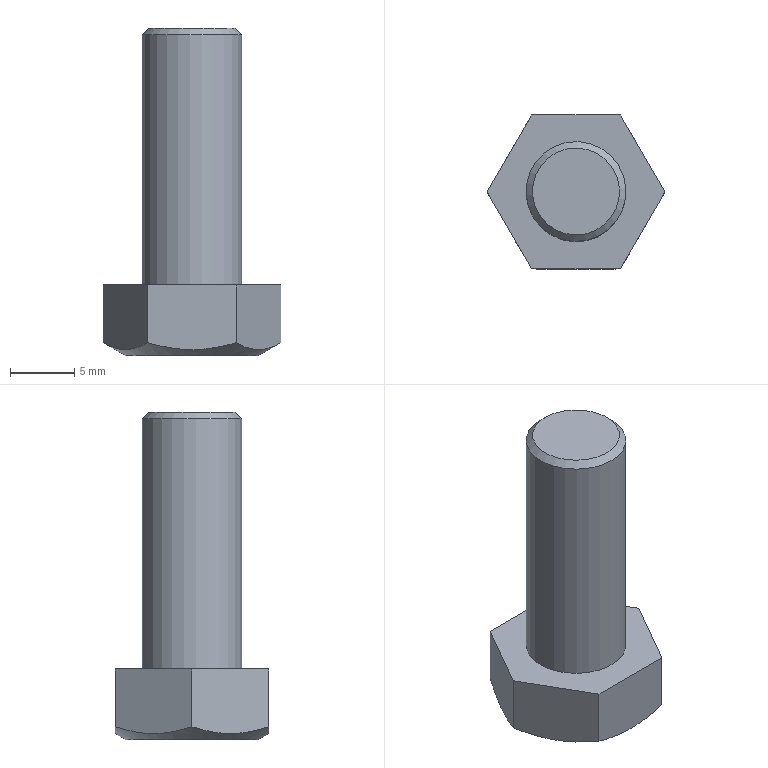Component | NX | BOLT_M8_X_20_2 | 1 solid | 12 faces | box 13.86 x 12 x 25.5 mm | volume 1621 mm3 | plane 9 | cone 2 | cylinder 1 | commonest cylinder face diameters 7.785 x1
STEP:
#1=CARTESIAN_POINT('',(0.,0.,0.));
#2=DIRECTION('',(0.,0.,1.));
#3=DIRECTION('',(1.,0.,0.));
#4=AXIS2_PLACEMENT_3D('',#1,#2,#3);
#5=CARTESIAN_POINT('',(-10.196,-39.311,-58.));
#6=VERTEX_POINT('',#5);
#7=CARTESIAN_POINT('',(-8.5,-36.373,-58.));
#8=DIRECTION('',(0.,0.,1.));
#9=DIRECTION('',(-0.5,-0.866,0.));
#10=AXIS2_PLACEMENT_3D('',#7,#8,#9);
#11=CIRCLE('',#10,3.393);
#12=CARTESIAN_POINT('',(-8.5,-36.373,-58.));
#13=DIRECTION('',(0.,0.,1.));
#14=DIRECTION('',(-0.5,-0.866,0.));
#15=AXIS2_PLACEMENT_3D('',#12,#13,#14);
#16=PLANE('',#15);
#17=CARTESIAN_POINT('',(0.,0.));
#18=DIRECTION('',(1.,-0.));
#19=AXIS2_PLACEMENT_2D('',#17,#18);
#20=CIRCLE('',#19,3.393);
#21=(GEOMETRIC_REPRESENTATION_CONTEXT(2)PARAMETRIC_REPRESENTATION_CONTEXT()REPRESENTATION_CONTEXT('',''));
#22=DEFINITIONAL_REPRESENTATION('',(#20),#21);
#23=PCURVE('',#16,#22);
#24=CARTESIAN_POINT('',(-8.5,-36.373,-58.5));
#25=DIRECTION('',(0.,0.,-1.));
#26=DIRECTION('',(0.5,0.866,0.));
#27=AXIS2_PLACEMENT_3D('',#24,#25,#26);
#28=CONICAL_SURFACE('',#27,3.893,0.7854);
#29=CARTESIAN_POINT('',(9.425,-0.5));
#30=DIRECTION('',(-1.,0.));
#31=VECTOR('',#30,1.);
#32=LINE('',#29,#31);
#33=(GEOMETRIC_REPRESENTATION_CONTEXT(2)PARAMETRIC_REPRESENTATION_CONTEXT()REPRESENTATION_CONTEXT('',''));
#34=DEFINITIONAL_REPRESENTATION('',(#32),#33);
#35=PCURVE('',#28,#34);
#36=SURFACE_CURVE('',#11,(#23,#35),.PCURVE_S1.);
#37=EDGE_CURVE('',#6,#6,#36,.T.);
#38=ORIENTED_EDGE('',*,*,#37,.T.);
#39=EDGE_LOOP('',(#38));
#40=FACE_BOUND('',#39,.T.);
#41=ADVANCED_FACE('',(#40),#16,.T.);
#42=CARTESIAN_POINT('',(-10.446,-39.744,-58.5));
#43=VERTEX_POINT('',#42);
#44=CARTESIAN_POINT('',(-6.554,-33.002,-58.5));
#45=VERTEX_POINT('',#44);
#46=CARTESIAN_POINT('',(-8.5,-36.373,-58.5));
#47=DIRECTION('',(0.,0.,-1.));
#48=DIRECTION('',(-0.5,-0.866,0.));
#49=AXIS2_PLACEMENT_3D('',#46,#47,#48);
#50=CIRCLE('',#49,3.893);
#51=CARTESIAN_POINT('',(-8.5,-36.373,-58.));
#52=DIRECTION('',(0.,0.,-1.));
#53=DIRECTION('',(0.5,0.866,0.));
#54=AXIS2_PLACEMENT_3D('',#51,#52,#53);
#55=CYLINDRICAL_SURFACE('',#54,3.893);
#56=CARTESIAN_POINT('',(3.142,0.5));
#57=DIRECTION('',(1.,0.));
#58=VECTOR('',#57,1.);
#59=LINE('',#56,#58);
#60=(GEOMETRIC_REPRESENTATION_CONTEXT(2)PARAMETRIC_REPRESENTATION_CONTEXT()REPRESENTATION_CONTEXT('',''));
#61=DEFINITIONAL_REPRESENTATION('',(#59),#60);
#62=PCURVE('',#55,#61);
#63=CARTESIAN_POINT('',(3.142,0.));
#64=DIRECTION('',(1.,0.));
#65=VECTOR('',#64,1.);
#66=LINE('',#63,#65);
#67=(GEOMETRIC_REPRESENTATION_CONTEXT(2)PARAMETRIC_REPRESENTATION_CONTEXT()REPRESENTATION_CONTEXT('',''));
#68=DEFINITIONAL_REPRESENTATION('',(#66),#67);
#69=PCURVE('',#28,#68);
#70=SURFACE_CURVE('',#50,(#62,#69),.PCURVE_S1.);
#71=EDGE_CURVE('',#43,#45,#70,.T.);
#72=ORIENTED_EDGE('',*,*,#71,.T.);
#73=CARTESIAN_POINT('',(-6.554,-33.002,-78.));
#74=VERTEX_POINT('',#73);
#75=CARTESIAN_POINT('',(-6.554,-33.002,-58.5));
#76=CARTESIAN_POINT('',(-6.554,-33.002,-78.));
#77=B_SPLINE_CURVE_WITH_KNOTS('',1,(#75,#76),.UNSPECIFIED.,.F.,.F.,(2,2),(0.5,20.),.PIECEWISE_BEZIER_KNOTS.);
#78=CARTESIAN_POINT('',(6.283,0.));
#79=DIRECTION('',(0.,1.));
#80=VECTOR('',#79,1.);
#81=LINE('',#78,#80);
#82=(GEOMETRIC_REPRESENTATION_CONTEXT(2)PARAMETRIC_REPRESENTATION_CONTEXT()REPRESENTATION_CONTEXT('',''));
#83=DEFINITIONAL_REPRESENTATION('',(#81),#82);
#84=PCURVE('',#55,#83);
#85=CARTESIAN_POINT('',(0.,0.));
#86=DIRECTION('',(0.,1.));
#87=VECTOR('',#86,1.);
#88=LINE('',#85,#87);
#89=(GEOMETRIC_REPRESENTATION_CONTEXT(2)PARAMETRIC_REPRESENTATION_CONTEXT()REPRESENTATION_CONTEXT('',''));
#90=DEFINITIONAL_REPRESENTATION('',(#88),#89);
#91=PCURVE('',#55,#90);
#92=SEAM_CURVE('',#77,(#84,#91),.PCURVE_S1.);
#93=EDGE_CURVE('',#45,#74,#92,.T.);
#94=ORIENTED_EDGE('',*,*,#93,.T.);
#95=CARTESIAN_POINT('',(-8.5,-36.373,-78.));
#96=DIRECTION('',(0.,0.,1.));
#97=DIRECTION('',(0.5,0.866,0.));
#98=AXIS2_PLACEMENT_3D('',#95,#96,#97);
#99=CIRCLE('',#98,3.893);
#100=CARTESIAN_POINT('',(6.283,20.));
#101=DIRECTION('',(-1.,0.));
#102=VECTOR('',#101,1.);
#103=LINE('',#100,#102);
#104=(GEOMETRIC_REPRESENTATION_CONTEXT(2)PARAMETRIC_REPRESENTATION_CONTEXT()REPRESENTATION_CONTEXT('',''));
#105=DEFINITIONAL_REPRESENTATION('',(#103),#104);
#106=PCURVE('',#55,#105);
#107=CARTESIAN_POINT('',(-8.5,-36.373,-78.));
#108=DIRECTION('',(0.,0.,1.));
#109=DIRECTION('',(-0.5,-0.866,0.));
#110=AXIS2_PLACEMENT_3D('',#107,#108,#109);
#111=PLANE('',#110);
#112=CARTESIAN_POINT('',(0.,0.));
#113=DIRECTION('',(-1.,0.));
#114=AXIS2_PLACEMENT_2D('',#112,#113);
#115=CIRCLE('',#114,3.893);
#116=(GEOMETRIC_REPRESENTATION_CONTEXT(2)PARAMETRIC_REPRESENTATION_CONTEXT()REPRESENTATION_CONTEXT('',''));
#117=DEFINITIONAL_REPRESENTATION('',(#115),#116);
#118=PCURVE('',#111,#117);
#119=SURFACE_CURVE('',#99,(#106,#118),.PCURVE_S1.);
#120=EDGE_CURVE('',#74,#74,#119,.T.);
#121=ORIENTED_EDGE('',*,*,#120,.T.);
#122=ORIENTED_EDGE('',*,*,#93,.F.);
#123=CARTESIAN_POINT('',(-8.5,-36.373,-58.5));
#124=DIRECTION('',(0.,0.,-1.));
#125=DIRECTION('',(-0.5,-0.866,0.));
#126=AXIS2_PLACEMENT_3D('',#123,#124,#125);
#127=CIRCLE('',#126,3.893);
#128=CARTESIAN_POINT('',(-3.142,0.5));
#129=DIRECTION('',(1.,0.));
#130=VECTOR('',#129,1.);
#131=LINE('',#128,#130);
#132=(GEOMETRIC_REPRESENTATION_CONTEXT(2)PARAMETRIC_REPRESENTATION_CONTEXT()REPRESENTATION_CONTEXT('',''));
#133=DEFINITIONAL_REPRESENTATION('',(#131),#132);
#134=PCURVE('',#55,#133);
#135=CARTESIAN_POINT('',(3.142,0.));
#136=DIRECTION('',(1.,-0.));
#137=VECTOR('',#136,1.);
#138=LINE('',#135,#137);
#139=(GEOMETRIC_REPRESENTATION_CONTEXT(2)PARAMETRIC_REPRESENTATION_CONTEXT()REPRESENTATION_CONTEXT('',''));
#140=DEFINITIONAL_REPRESENTATION('',(#138),#139);
#141=PCURVE('',#28,#140);
#142=SURFACE_CURVE('',#127,(#134,#141),.PCURVE_S1.);
#143=EDGE_CURVE('',#45,#43,#142,.T.);
#144=ORIENTED_EDGE('',*,*,#143,.T.);
#145=EDGE_LOOP('',(#72,#94,#121,#122,#144));
#146=FACE_BOUND('',#145,.T.);
#147=ADVANCED_FACE('',(#146),#55,.T.);
#148=CARTESIAN_POINT('',(-5.036,-30.373,-82.5));
#149=VERTEX_POINT('',#148);
#150=CARTESIAN_POINT('',(-1.572,-36.373,-82.5));
#151=VERTEX_POINT('',#150);
#152=CARTESIAN_POINT('',(-5.036,-30.373,-82.5));
#153=CARTESIAN_POINT('',(-4.47,-31.353,-82.827));
#154=CARTESIAN_POINT('',(-3.896,-32.347,-83.035));
#155=CARTESIAN_POINT('',(-2.718,-34.388,-83.037));
#156=CARTESIAN_POINT('',(-2.138,-35.392,-82.827));
#157=CARTESIAN_POINT('',(-1.572,-36.373,-82.5));
#158=B_SPLINE_CURVE_WITH_KNOTS('',3,(#152,#153,#154,#155,#156,#157),.UNSPECIFIED.,.F.,.F.,(4,2,4),(0.,0.5,1.),.UNSPECIFIED.);
#159=CARTESIAN_POINT('',(-1.572,-36.373,-83.5));
#160=DIRECTION('',(0.866,0.5,0.));
#161=DIRECTION('',(0.5,-0.866,0.));
#162=AXIS2_PLACEMENT_3D('',#159,#160,#161);
#163=PLANE('',#162);
#164=CARTESIAN_POINT('',(-6.928,-1.));
#165=CARTESIAN_POINT('',(-5.797,-0.6734));
#166=CARTESIAN_POINT('',(-4.649,-0.4649));
#167=CARTESIAN_POINT('',(-2.293,-0.4634));
#168=CARTESIAN_POINT('',(-1.133,-0.673));
#169=CARTESIAN_POINT('',(0.,-1.));
#170=B_SPLINE_CURVE_WITH_KNOTS('',3,(#164,#165,#166,#167,#168,#169),.UNSPECIFIED.,.F.,.F.,(4,2,4),(0.,0.5,1.),.UNSPECIFIED.);
#171=(GEOMETRIC_REPRESENTATION_CONTEXT(2)PARAMETRIC_REPRESENTATION_CONTEXT()REPRESENTATION_CONTEXT('',''));
#172=DEFINITIONAL_REPRESENTATION('',(#170),#171);
#173=PCURVE('',#163,#172);
#174=CARTESIAN_POINT('',(-8.5,-36.373,-83.5));
#175=DIRECTION('',(0.,0.,1.));
#176=DIRECTION('',(-0.5,-0.866,0.));
#177=AXIS2_PLACEMENT_3D('',#174,#175,#176);
#178=CONICAL_SURFACE('',#177,5.196,1.047);
#179=CARTESIAN_POINT('',(3.142,1.));
#180=CARTESIAN_POINT('',(3.129,0.9703));
#181=CARTESIAN_POINT('',(3.102,0.9129));
#182=CARTESIAN_POINT('',(3.061,0.8328));
#183=CARTESIAN_POINT('',(3.018,0.7594));
#184=CARTESIAN_POINT('',(2.973,0.6931));
#185=CARTESIAN_POINT('',(2.926,0.6342));
#186=CARTESIAN_POINT('',(2.878,0.5834));
#187=CARTESIAN_POINT('',(2.828,0.5409));
#188=CARTESIAN_POINT('',(2.777,0.5072));
#189=CARTESIAN_POINT('',(2.725,0.4827));
#190=CARTESIAN_POINT('',(2.673,0.4677));
#191=CARTESIAN_POINT('',(2.619,0.4624));
#192=CARTESIAN_POINT('',(2.566,0.4673));
#193=CARTESIAN_POINT('',(2.513,0.4819));
#194=CARTESIAN_POINT('',(2.46,0.5062));
#195=CARTESIAN_POINT('',(2.409,0.5398));
#196=CARTESIAN_POINT('',(2.359,0.5823));
#197=CARTESIAN_POINT('',(2.311,0.6332));
#198=CARTESIAN_POINT('',(2.264,0.6922));
#199=CARTESIAN_POINT('',(2.218,0.7588));
#200=CARTESIAN_POINT('',(2.175,0.8325));
#201=CARTESIAN_POINT('',(2.134,0.9127));
#202=CARTESIAN_POINT('',(2.107,0.9703));
#203=CARTESIAN_POINT('',(2.094,1.));
#204=B_SPLINE_CURVE_WITH_KNOTS('',3,(#179,#180,#181,#182,#183,#184,#185,#186,#187,#188,#189,#190,#191,#192,#193,#194,#195,#196,#197,#198,#199,#200,#201,#202,#203),.UNSPECIFIED.,.F.,.F.,(4,1,1,1,1,1,1,1,1,1,1,1,1,1,1,1,1,1,1,1,1,1,4),(0.,0.04545,0.09091,0.1364,0.1818,0.2273,0.2727,0.3182,0.3636,0.4091,0.4545,0.5,0.5455,0.5909,0.6364,0.6818,0.7273,0.7727,0.8182,0.8636,0.9091,0.9545,1.),.QUASI_UNIFORM_KNOTS.);
#205=(GEOMETRIC_REPRESENTATION_CONTEXT(2)PARAMETRIC_REPRESENTATION_CONTEXT()REPRESENTATION_CONTEXT('',''));
#206=DEFINITIONAL_REPRESENTATION('',(#204),#205);
#207=PCURVE('',#178,#206);
#208=SURFACE_CURVE('',#158,(#173,#207),.PCURVE_S1.);
#209=EDGE_CURVE('',#149,#151,#208,.T.);
#210=ORIENTED_EDGE('',*,*,#209,.F.);
#211=CARTESIAN_POINT('',(-5.036,-30.373,-78.));
#212=VERTEX_POINT('',#211);
#213=CARTESIAN_POINT('',(-5.036,-30.373,-83.5));
#214=DIRECTION('',(0.,0.,1.));
#215=VECTOR('',#214,1.);
#216=LINE('',#213,#215);
#217=CARTESIAN_POINT('',(-6.928,0.));
#218=DIRECTION('',(0.,-1.));
#219=VECTOR('',#218,1.);
#220=LINE('',#217,#219);
#221=(GEOMETRIC_REPRESENTATION_CONTEXT(2)PARAMETRIC_REPRESENTATION_CONTEXT()REPRESENTATION_CONTEXT('',''));
#222=DEFINITIONAL_REPRESENTATION('',(#220),#221);
#223=PCURVE('',#163,#222);
#224=CARTESIAN_POINT('',(-5.036,-30.373,-83.5));
#225=DIRECTION('',(0.,1.,0.));
#226=DIRECTION('',(1.,-0.,0.));
#227=AXIS2_PLACEMENT_3D('',#224,#225,#226);
#228=PLANE('',#227);
#229=CARTESIAN_POINT('',(0.,0.));
#230=DIRECTION('',(0.,-1.));
#231=VECTOR('',#230,1.);
#232=LINE('',#229,#231);
#233=(GEOMETRIC_REPRESENTATION_CONTEXT(2)PARAMETRIC_REPRESENTATION_CONTEXT()REPRESENTATION_CONTEXT('',''));
#234=DEFINITIONAL_REPRESENTATION('',(#232),#233);
#235=PCURVE('',#228,#234);
#236=SURFACE_CURVE('',#216,(#223,#235),.PCURVE_S1.);
#237=EDGE_CURVE('',#149,#212,#236,.T.);
#238=ORIENTED_EDGE('',*,*,#237,.T.);
#239=CARTESIAN_POINT('',(-1.572,-36.373,-78.));
#240=VERTEX_POINT('',#239);
#241=CARTESIAN_POINT('',(-1.572,-36.373,-78.));
#242=DIRECTION('',(-0.5,0.866,0.));
#243=VECTOR('',#242,1.);
#244=LINE('',#241,#243);
#245=CARTESIAN_POINT('',(0.,-5.5));
#246=DIRECTION('',(-1.,0.));
#247=VECTOR('',#246,1.);
#248=LINE('',#245,#247);
#249=(GEOMETRIC_REPRESENTATION_CONTEXT(2)PARAMETRIC_REPRESENTATION_CONTEXT()REPRESENTATION_CONTEXT('',''));
#250=DEFINITIONAL_REPRESENTATION('',(#248),#249);
#251=PCURVE('',#163,#250);
#252=CARTESIAN_POINT('',(-3.464,6.));
#253=DIRECTION('',(-0.5,-0.866));
#254=VECTOR('',#253,1.);
#255=LINE('',#252,#254);
#256=(GEOMETRIC_REPRESENTATION_CONTEXT(2)PARAMETRIC_REPRESENTATION_CONTEXT()REPRESENTATION_CONTEXT('',''));
#257=DEFINITIONAL_REPRESENTATION('',(#255),#256);
#258=PCURVE('',#111,#257);
#259=SURFACE_CURVE('',#244,(#251,#258),.PCURVE_S1.);
#260=EDGE_CURVE('',#240,#212,#259,.T.);
#261=ORIENTED_EDGE('',*,*,#260,.F.);
#262=CARTESIAN_POINT('',(-1.572,-36.373,-83.5));
#263=DIRECTION('',(0.,0.,1.));
#264=VECTOR('',#263,1.);
#265=LINE('',#262,#264);
#266=CARTESIAN_POINT('',(0.,0.));
#267=DIRECTION('',(0.,-1.));
#268=VECTOR('',#267,1.);
#269=LINE('',#266,#268);
#270=(GEOMETRIC_REPRESENTATION_CONTEXT(2)PARAMETRIC_REPRESENTATION_CONTEXT()REPRESENTATION_CONTEXT('',''));
#271=DEFINITIONAL_REPRESENTATION('',(#269),#270);
#272=PCURVE('',#163,#271);
#273=CARTESIAN_POINT('',(-5.036,-42.373,-83.5));
#274=DIRECTION('',(0.866,-0.5,0.));
#275=DIRECTION('',(0.,0.,-1.));
#276=AXIS2_PLACEMENT_3D('',#273,#274,#275);
#277=PLANE('',#276);
#278=CARTESIAN_POINT('',(0.,6.928));
#279=DIRECTION('',(-1.,0.));
#280=VECTOR('',#279,1.);
#281=LINE('',#278,#280);
#282=(GEOMETRIC_REPRESENTATION_CONTEXT(2)PARAMETRIC_REPRESENTATION_CONTEXT()REPRESENTATION_CONTEXT('',''));
#283=DEFINITIONAL_REPRESENTATION('',(#281),#282);
#284=PCURVE('',#277,#283);
#285=SURFACE_CURVE('',#265,(#272,#284),.PCURVE_S1.);
#286=EDGE_CURVE('',#151,#240,#285,.T.);
#287=ORIENTED_EDGE('',*,*,#286,.F.);
#288=EDGE_LOOP('',(#210,#238,#261,#287));
#289=FACE_BOUND('',#288,.T.);
#290=ADVANCED_FACE('',(#289),#163,.T.);
#291=CARTESIAN_POINT('',(-11.964,-30.373,-82.5));
#292=VERTEX_POINT('',#291);
#293=CARTESIAN_POINT('',(-11.964,-30.373,-82.5));
#294=CARTESIAN_POINT('',(-10.833,-30.373,-82.827));
#295=CARTESIAN_POINT('',(-9.685,-30.373,-83.035));
#296=CARTESIAN_POINT('',(-7.329,-30.373,-83.037));
#297=CARTESIAN_POINT('',(-6.169,-30.373,-82.827));
#298=CARTESIAN_POINT('',(-5.036,-30.373,-82.5));
#299=B_SPLINE_CURVE_WITH_KNOTS('',3,(#293,#294,#295,#296,#297,#298),.UNSPECIFIED.,.F.,.F.,(4,2,4),(0.,0.5,1.),.UNSPECIFIED.);
#300=CARTESIAN_POINT('',(-6.928,-1.));
#301=CARTESIAN_POINT('',(-5.797,-0.6734));
#302=CARTESIAN_POINT('',(-4.649,-0.4649));
#303=CARTESIAN_POINT('',(-2.293,-0.4634));
#304=CARTESIAN_POINT('',(-1.133,-0.673));
#305=CARTESIAN_POINT('',(0.,-1.));
#306=B_SPLINE_CURVE_WITH_KNOTS('',3,(#300,#301,#302,#303,#304,#305),.UNSPECIFIED.,.F.,.F.,(4,2,4),(0.,0.5,1.),.UNSPECIFIED.);
#307=(GEOMETRIC_REPRESENTATION_CONTEXT(2)PARAMETRIC_REPRESENTATION_CONTEXT()REPRESENTATION_CONTEXT('',''));
#308=DEFINITIONAL_REPRESENTATION('',(#306),#307);
#309=PCURVE('',#228,#308);
#310=CARTESIAN_POINT('',(4.189,1.));
#311=CARTESIAN_POINT('',(4.176,0.9703));
#312=CARTESIAN_POINT('',(4.15,0.9129));
#313=CARTESIAN_POINT('',(4.108,0.8328));
#314=CARTESIAN_POINT('',(4.065,0.7594));
#315=CARTESIAN_POINT('',(4.02,0.6931));
#316=CARTESIAN_POINT('',(3.974,0.6342));
#317=CARTESIAN_POINT('',(3.925,0.5834));
#318=CARTESIAN_POINT('',(3.876,0.5409));
#319=CARTESIAN_POINT('',(3.825,0.5072));
#320=CARTESIAN_POINT('',(3.773,0.4827));
#321=CARTESIAN_POINT('',(3.72,0.4677));
#322=CARTESIAN_POINT('',(3.666,0.4624));
#323=CARTESIAN_POINT('',(3.613,0.4673));
#324=CARTESIAN_POINT('',(3.56,0.4819));
#325=CARTESIAN_POINT('',(3.507,0.5062));
#326=CARTESIAN_POINT('',(3.456,0.5398));
#327=CARTESIAN_POINT('',(3.406,0.5823));
#328=CARTESIAN_POINT('',(3.358,0.6332));
#329=CARTESIAN_POINT('',(3.311,0.6922));
#330=CARTESIAN_POINT('',(3.266,0.7588));
#331=CARTESIAN_POINT('',(3.222,0.8325));
#332=CARTESIAN_POINT('',(3.181,0.9127));
#333=CARTESIAN_POINT('',(3.154,0.9703));
#334=CARTESIAN_POINT('',(3.142,1.));
#335=B_SPLINE_CURVE_WITH_KNOTS('',3,(#310,#311,#312,#313,#314,#315,#316,#317,#318,#319,#320,#321,#322,#323,#324,#325,#326,#327,#328,#329,#330,#331,#332,#333,#334),.UNSPECIFIED.,.F.,.F.,(4,1,1,1,1,1,1,1,1,1,1,1,1,1,1,1,1,1,1,1,1,1,4),(0.,0.04545,0.09091,0.1364,0.1818,0.2273,0.2727,0.3182,0.3636,0.4091,0.4545,0.5,0.5455,0.5909,0.6364,0.6818,0.7273,0.7727,0.8182,0.8636,0.9091,0.9545,1.),.QUASI_UNIFORM_KNOTS.);
#336=(GEOMETRIC_REPRESENTATION_CONTEXT(2)PARAMETRIC_REPRESENTATION_CONTEXT()REPRESENTATION_CONTEXT('',''));
#337=DEFINITIONAL_REPRESENTATION('',(#335),#336);
#338=PCURVE('',#178,#337);
#339=SURFACE_CURVE('',#299,(#309,#338),.PCURVE_S1.);
#340=EDGE_CURVE('',#292,#149,#339,.T.);
#341=ORIENTED_EDGE('',*,*,#340,.F.);
#342=CARTESIAN_POINT('',(-11.964,-30.373,-78.));
#343=VERTEX_POINT('',#342);
#344=CARTESIAN_POINT('',(-11.964,-30.373,-83.5));
#345=DIRECTION('',(0.,0.,1.));
#346=VECTOR('',#345,1.);
#347=LINE('',#344,#346);
#348=CARTESIAN_POINT('',(-6.928,0.));
#349=DIRECTION('',(0.,-1.));
#350=VECTOR('',#349,1.);
#351=LINE('',#348,#350);
#352=(GEOMETRIC_REPRESENTATION_CONTEXT(2)PARAMETRIC_REPRESENTATION_CONTEXT()REPRESENTATION_CONTEXT('',''));
#353=DEFINITIONAL_REPRESENTATION('',(#351),#352);
#354=PCURVE('',#228,#353);
#355=CARTESIAN_POINT('',(-11.964,-30.373,-83.5));
#356=DIRECTION('',(-0.866,0.5,0.));
#357=DIRECTION('',(0.5,0.866,0.));
#358=AXIS2_PLACEMENT_3D('',#355,#356,#357);
#359=PLANE('',#358);
#360=CARTESIAN_POINT('',(0.,0.));
#361=DIRECTION('',(0.,-1.));
#362=VECTOR('',#361,1.);
#363=LINE('',#360,#362);
#364=(GEOMETRIC_REPRESENTATION_CONTEXT(2)PARAMETRIC_REPRESENTATION_CONTEXT()REPRESENTATION_CONTEXT('',''));
#365=DEFINITIONAL_REPRESENTATION('',(#363),#364);
#366=PCURVE('',#359,#365);
#367=SURFACE_CURVE('',#347,(#354,#366),.PCURVE_S1.);
#368=EDGE_CURVE('',#292,#343,#367,.T.);
#369=ORIENTED_EDGE('',*,*,#368,.T.);
#370=CARTESIAN_POINT('',(-5.036,-30.373,-78.));
#371=DIRECTION('',(-1.,0.,0.));
#372=VECTOR('',#371,1.);
#373=LINE('',#370,#372);
#374=CARTESIAN_POINT('',(0.,-5.5));
#375=DIRECTION('',(-1.,0.));
#376=VECTOR('',#375,1.);
#377=LINE('',#374,#376);
#378=(GEOMETRIC_REPRESENTATION_CONTEXT(2)PARAMETRIC_REPRESENTATION_CONTEXT()REPRESENTATION_CONTEXT('',''));
#379=DEFINITIONAL_REPRESENTATION('',(#377),#378);
#380=PCURVE('',#228,#379);
#381=CARTESIAN_POINT('',(-6.928,-0.));
#382=DIRECTION('',(0.5,-0.866));
#383=VECTOR('',#382,1.);
#384=LINE('',#381,#383);
#385=(GEOMETRIC_REPRESENTATION_CONTEXT(2)PARAMETRIC_REPRESENTATION_CONTEXT()REPRESENTATION_CONTEXT('',''));
#386=DEFINITIONAL_REPRESENTATION('',(#384),#385);
#387=PCURVE('',#111,#386);
#388=SURFACE_CURVE('',#373,(#380,#387),.PCURVE_S1.);
#389=EDGE_CURVE('',#212,#343,#388,.T.);
#390=ORIENTED_EDGE('',*,*,#389,.F.);
#391=ORIENTED_EDGE('',*,*,#237,.F.);
#392=EDGE_LOOP('',(#341,#369,#390,#391));
#393=FACE_BOUND('',#392,.T.);
#394=ADVANCED_FACE('',(#393),#228,.T.);
#395=CARTESIAN_POINT('',(-15.428,-36.373,-82.5));
#396=VERTEX_POINT('',#395);
#397=CARTESIAN_POINT('',(-15.428,-36.373,-82.5));
#398=CARTESIAN_POINT('',(-14.865,-35.397,-82.825));
#399=CARTESIAN_POINT('',(-14.281,-34.386,-83.036));
#400=CARTESIAN_POINT('',(-13.11,-32.358,-83.036));
#401=CARTESIAN_POINT('',(-12.524,-31.343,-82.823));
#402=CARTESIAN_POINT('',(-11.964,-30.373,-82.5));
#403=B_SPLINE_CURVE_WITH_KNOTS('',3,(#397,#398,#399,#400,#401,#402),.UNSPECIFIED.,.F.,.F.,(4,2,4),(0.,0.5,1.),.UNSPECIFIED.);
#404=CARTESIAN_POINT('',(-6.928,-1.));
#405=CARTESIAN_POINT('',(-5.801,-0.6747));
#406=CARTESIAN_POINT('',(-4.634,-0.464));
#407=CARTESIAN_POINT('',(-2.292,-0.4642));
#408=CARTESIAN_POINT('',(-1.12,-0.6767));
#409=CARTESIAN_POINT('',(0.,-1.));
#410=B_SPLINE_CURVE_WITH_KNOTS('',3,(#404,#405,#406,#407,#408,#409),.UNSPECIFIED.,.F.,.F.,(4,2,4),(0.,0.5,1.),.UNSPECIFIED.);
#411=(GEOMETRIC_REPRESENTATION_CONTEXT(2)PARAMETRIC_REPRESENTATION_CONTEXT()REPRESENTATION_CONTEXT('',''));
#412=DEFINITIONAL_REPRESENTATION('',(#410),#411);
#413=PCURVE('',#359,#412);
#414=CARTESIAN_POINT('',(5.236,1.));
#415=CARTESIAN_POINT('',(5.223,0.9704));
#416=CARTESIAN_POINT('',(5.197,0.9131));
#417=CARTESIAN_POINT('',(5.156,0.833));
#418=CARTESIAN_POINT('',(5.112,0.7594));
#419=CARTESIAN_POINT('',(5.067,0.6928));
#420=CARTESIAN_POINT('',(5.02,0.6338));
#421=CARTESIAN_POINT('',(4.972,0.5827));
#422=CARTESIAN_POINT('',(4.922,0.5402));
#423=CARTESIAN_POINT('',(4.87,0.5065));
#424=CARTESIAN_POINT('',(4.818,0.4822));
#425=CARTESIAN_POINT('',(4.765,0.4674));
#426=CARTESIAN_POINT('',(4.712,0.4624));
#427=CARTESIAN_POINT('',(4.659,0.4675));
#428=CARTESIAN_POINT('',(4.606,0.4823));
#429=CARTESIAN_POINT('',(4.554,0.5068));
#430=CARTESIAN_POINT('',(4.503,0.5406));
#431=CARTESIAN_POINT('',(4.453,0.5833));
#432=CARTESIAN_POINT('',(4.404,0.6345));
#433=CARTESIAN_POINT('',(4.357,0.6936));
#434=CARTESIAN_POINT('',(4.312,0.7602));
#435=CARTESIAN_POINT('',(4.269,0.8337));
#436=CARTESIAN_POINT('',(4.228,0.9136));
#437=CARTESIAN_POINT('',(4.202,0.9706));
#438=CARTESIAN_POINT('',(4.189,1.));
#439=B_SPLINE_CURVE_WITH_KNOTS('',3,(#414,#415,#416,#417,#418,#419,#420,#421,#422,#423,#424,#425,#426,#427,#428,#429,#430,#431,#432,#433,#434,#435,#436,#437,#438),.UNSPECIFIED.,.F.,.F.,(4,1,1,1,1,1,1,1,1,1,1,1,1,1,1,1,1,1,1,1,1,1,4),(0.,0.04545,0.09091,0.1364,0.1818,0.2273,0.2727,0.3182,0.3636,0.4091,0.4545,0.5,0.5455,0.5909,0.6364,0.6818,0.7273,0.7727,0.8182,0.8636,0.9091,0.9545,1.),.QUASI_UNIFORM_KNOTS.);
#440=(GEOMETRIC_REPRESENTATION_CONTEXT(2)PARAMETRIC_REPRESENTATION_CONTEXT()REPRESENTATION_CONTEXT('',''));
#441=DEFINITIONAL_REPRESENTATION('',(#439),#440);
#442=PCURVE('',#178,#441);
#443=SURFACE_CURVE('',#403,(#413,#442),.PCURVE_S1.);
#444=EDGE_CURVE('',#396,#292,#443,.T.);
#445=ORIENTED_EDGE('',*,*,#444,.F.);
#446=CARTESIAN_POINT('',(-15.428,-36.373,-78.));
#447=VERTEX_POINT('',#446);
#448=CARTESIAN_POINT('',(-15.428,-36.373,-83.5));
#449=DIRECTION('',(0.,0.,1.));
#450=VECTOR('',#449,1.);
#451=LINE('',#448,#450);
#452=CARTESIAN_POINT('',(-6.928,0.));
#453=DIRECTION('',(0.,-1.));
#454=VECTOR('',#453,1.);
#455=LINE('',#452,#454);
#456=(GEOMETRIC_REPRESENTATION_CONTEXT(2)PARAMETRIC_REPRESENTATION_CONTEXT()REPRESENTATION_CONTEXT('',''));
#457=DEFINITIONAL_REPRESENTATION('',(#455),#456);
#458=PCURVE('',#359,#457);
#459=CARTESIAN_POINT('',(-15.428,-36.373,-83.5));
#460=DIRECTION('',(-0.866,-0.5,0.));
#461=DIRECTION('',(-0.5,0.866,0.));
#462=AXIS2_PLACEMENT_3D('',#459,#460,#461);
#463=PLANE('',#462);
#464=CARTESIAN_POINT('',(0.,0.));
#465=DIRECTION('',(0.,-1.));
#466=VECTOR('',#465,1.);
#467=LINE('',#464,#466);
#468=(GEOMETRIC_REPRESENTATION_CONTEXT(2)PARAMETRIC_REPRESENTATION_CONTEXT()REPRESENTATION_CONTEXT('',''));
#469=DEFINITIONAL_REPRESENTATION('',(#467),#468);
#470=PCURVE('',#463,#469);
#471=SURFACE_CURVE('',#451,(#458,#470),.PCURVE_S1.);
#472=EDGE_CURVE('',#396,#447,#471,.T.);
#473=ORIENTED_EDGE('',*,*,#472,.T.);
#474=CARTESIAN_POINT('',(-11.964,-30.373,-78.));
#475=DIRECTION('',(-0.5,-0.866,0.));
#476=VECTOR('',#475,1.);
#477=LINE('',#474,#476);
#478=CARTESIAN_POINT('',(0.,-5.5));
#479=DIRECTION('',(-1.,0.));
#480=VECTOR('',#479,1.);
#481=LINE('',#478,#480);
#482=(GEOMETRIC_REPRESENTATION_CONTEXT(2)PARAMETRIC_REPRESENTATION_CONTEXT()REPRESENTATION_CONTEXT('',''));
#483=DEFINITIONAL_REPRESENTATION('',(#481),#482);
#484=PCURVE('',#359,#483);
#485=CARTESIAN_POINT('',(-3.464,-6.));
#486=DIRECTION('',(1.,0.));
#487=VECTOR('',#486,1.);
#488=LINE('',#485,#487);
#489=(GEOMETRIC_REPRESENTATION_CONTEXT(2)PARAMETRIC_REPRESENTATION_CONTEXT()REPRESENTATION_CONTEXT('',''));
#490=DEFINITIONAL_REPRESENTATION('',(#488),#489);
#491=PCURVE('',#111,#490);
#492=SURFACE_CURVE('',#477,(#484,#491),.PCURVE_S1.);
#493=EDGE_CURVE('',#343,#447,#492,.T.);
#494=ORIENTED_EDGE('',*,*,#493,.F.);
#495=ORIENTED_EDGE('',*,*,#368,.F.);
#496=EDGE_LOOP('',(#445,#473,#494,#495));
#497=FACE_BOUND('',#496,.T.);
#498=ADVANCED_FACE('',(#497),#359,.T.);
#499=CARTESIAN_POINT('',(-11.964,-42.373,-82.5));
#500=VERTEX_POINT('',#499);
#501=CARTESIAN_POINT('',(-11.964,-42.373,-82.5));
#502=CARTESIAN_POINT('',(-12.53,-41.393,-82.827));
#503=CARTESIAN_POINT('',(-13.104,-40.399,-83.035));
#504=CARTESIAN_POINT('',(-14.282,-38.359,-83.037));
#505=CARTESIAN_POINT('',(-14.862,-37.354,-82.827));
#506=CARTESIAN_POINT('',(-15.428,-36.373,-82.5));
#507=B_SPLINE_CURVE_WITH_KNOTS('',3,(#501,#502,#503,#504,#505,#506),.UNSPECIFIED.,.F.,.F.,(4,2,4),(0.,0.5,1.),.UNSPECIFIED.);
#508=CARTESIAN_POINT('',(-6.928,-1.));
#509=CARTESIAN_POINT('',(-5.797,-0.6734));
#510=CARTESIAN_POINT('',(-4.649,-0.4649));
#511=CARTESIAN_POINT('',(-2.293,-0.4634));
#512=CARTESIAN_POINT('',(-1.133,-0.673));
#513=CARTESIAN_POINT('',(0.,-1.));
#514=B_SPLINE_CURVE_WITH_KNOTS('',3,(#508,#509,#510,#511,#512,#513),.UNSPECIFIED.,.F.,.F.,(4,2,4),(0.,0.5,1.),.UNSPECIFIED.);
#515=(GEOMETRIC_REPRESENTATION_CONTEXT(2)PARAMETRIC_REPRESENTATION_CONTEXT()REPRESENTATION_CONTEXT('',''));
#516=DEFINITIONAL_REPRESENTATION('',(#514),#515);
#517=PCURVE('',#463,#516);
#518=CARTESIAN_POINT('',(6.283,1.));
#519=CARTESIAN_POINT('',(6.27,0.9703));
#520=CARTESIAN_POINT('',(6.244,0.9129));
#521=CARTESIAN_POINT('',(6.203,0.8328));
#522=CARTESIAN_POINT('',(6.16,0.7594));
#523=CARTESIAN_POINT('',(6.115,0.6931));
#524=CARTESIAN_POINT('',(6.068,0.6342));
#525=CARTESIAN_POINT('',(6.02,0.5834));
#526=CARTESIAN_POINT('',(5.97,0.5409));
#527=CARTESIAN_POINT('',(5.919,0.5072));
#528=CARTESIAN_POINT('',(5.867,0.4827));
#529=CARTESIAN_POINT('',(5.814,0.4677));
#530=CARTESIAN_POINT('',(5.761,0.4624));
#531=CARTESIAN_POINT('',(5.707,0.4673));
#532=CARTESIAN_POINT('',(5.654,0.4819));
#533=CARTESIAN_POINT('',(5.602,0.5062));
#534=CARTESIAN_POINT('',(5.551,0.5398));
#535=CARTESIAN_POINT('',(5.501,0.5823));
#536=CARTESIAN_POINT('',(5.452,0.6332));
#537=CARTESIAN_POINT('',(5.405,0.6922));
#538=CARTESIAN_POINT('',(5.36,0.7588));
#539=CARTESIAN_POINT('',(5.317,0.8325));
#540=CARTESIAN_POINT('',(5.275,0.9127));
#541=CARTESIAN_POINT('',(5.249,0.9703));
#542=CARTESIAN_POINT('',(5.236,1.));
#543=B_SPLINE_CURVE_WITH_KNOTS('',3,(#518,#519,#520,#521,#522,#523,#524,#525,#526,#527,#528,#529,#530,#531,#532,#533,#534,#535,#536,#537,#538,#539,#540,#541,#542),.UNSPECIFIED.,.F.,.F.,(4,1,1,1,1,1,1,1,1,1,1,1,1,1,1,1,1,1,1,1,1,1,4),(0.,0.04545,0.09091,0.1364,0.1818,0.2273,0.2727,0.3182,0.3636,0.4091,0.4545,0.5,0.5455,0.5909,0.6364,0.6818,0.7273,0.7727,0.8182,0.8636,0.9091,0.9545,1.),.QUASI_UNIFORM_KNOTS.);
#544=(GEOMETRIC_REPRESENTATION_CONTEXT(2)PARAMETRIC_REPRESENTATION_CONTEXT()REPRESENTATION_CONTEXT('',''));
#545=DEFINITIONAL_REPRESENTATION('',(#543),#544);
#546=PCURVE('',#178,#545);
#547=SURFACE_CURVE('',#507,(#517,#546),.PCURVE_S1.);
#548=EDGE_CURVE('',#500,#396,#547,.T.);
#549=ORIENTED_EDGE('',*,*,#548,.F.);
#550=CARTESIAN_POINT('',(-11.964,-42.373,-78.));
#551=VERTEX_POINT('',#550);
#552=CARTESIAN_POINT('',(-11.964,-42.373,-83.5));
#553=DIRECTION('',(0.,0.,1.));
#554=VECTOR('',#553,1.);
#555=LINE('',#552,#554);
#556=CARTESIAN_POINT('',(-6.928,0.));
#557=DIRECTION('',(0.,-1.));
#558=VECTOR('',#557,1.);
#559=LINE('',#556,#558);
#560=(GEOMETRIC_REPRESENTATION_CONTEXT(2)PARAMETRIC_REPRESENTATION_CONTEXT()REPRESENTATION_CONTEXT('',''));
#561=DEFINITIONAL_REPRESENTATION('',(#559),#560);
#562=PCURVE('',#463,#561);
#563=CARTESIAN_POINT('',(-11.964,-42.373,-83.5));
#564=DIRECTION('',(-0.,-1.,0.));
#565=DIRECTION('',(-1.,0.,0.));
#566=AXIS2_PLACEMENT_3D('',#563,#564,#565);
#567=PLANE('',#566);
#568=CARTESIAN_POINT('',(0.,0.));
#569=DIRECTION('',(0.,-1.));
#570=VECTOR('',#569,1.);
#571=LINE('',#568,#570);
#572=(GEOMETRIC_REPRESENTATION_CONTEXT(2)PARAMETRIC_REPRESENTATION_CONTEXT()REPRESENTATION_CONTEXT('',''));
#573=DEFINITIONAL_REPRESENTATION('',(#571),#572);
#574=PCURVE('',#567,#573);
#575=SURFACE_CURVE('',#555,(#562,#574),.PCURVE_S1.);
#576=EDGE_CURVE('',#500,#551,#575,.T.);
#577=ORIENTED_EDGE('',*,*,#576,.T.);
#578=CARTESIAN_POINT('',(-15.428,-36.373,-78.));
#579=DIRECTION('',(0.5,-0.866,0.));
#580=VECTOR('',#579,1.);
#581=LINE('',#578,#580);
#582=CARTESIAN_POINT('',(0.,-5.5));
#583=DIRECTION('',(-1.,0.));
#584=VECTOR('',#583,1.);
#585=LINE('',#582,#584);
#586=(GEOMETRIC_REPRESENTATION_CONTEXT(2)PARAMETRIC_REPRESENTATION_CONTEXT()REPRESENTATION_CONTEXT('',''));
#587=DEFINITIONAL_REPRESENTATION('',(#585),#586);
#588=PCURVE('',#463,#587);
#589=CARTESIAN_POINT('',(3.464,-6.));
#590=DIRECTION('',(0.5,0.866));
#591=VECTOR('',#590,1.);
#592=LINE('',#589,#591);
#593=(GEOMETRIC_REPRESENTATION_CONTEXT(2)PARAMETRIC_REPRESENTATION_CONTEXT()REPRESENTATION_CONTEXT('',''));
#594=DEFINITIONAL_REPRESENTATION('',(#592),#593);
#595=PCURVE('',#111,#594);
#596=SURFACE_CURVE('',#581,(#588,#595),.PCURVE_S1.);
#597=EDGE_CURVE('',#447,#551,#596,.T.);
#598=ORIENTED_EDGE('',*,*,#597,.F.);
#599=ORIENTED_EDGE('',*,*,#472,.F.);
#600=EDGE_LOOP('',(#549,#577,#598,#599));
#601=FACE_BOUND('',#600,.T.);
#602=ADVANCED_FACE('',(#601),#463,.T.);
#603=CARTESIAN_POINT('',(-5.036,-42.373,-82.5));
#604=VERTEX_POINT('',#603);
#605=CARTESIAN_POINT('',(-5.036,-42.373,-82.5));
#606=CARTESIAN_POINT('',(-6.167,-42.373,-82.827));
#607=CARTESIAN_POINT('',(-7.315,-42.373,-83.035));
#608=CARTESIAN_POINT('',(-9.671,-42.373,-83.037));
#609=CARTESIAN_POINT('',(-10.831,-42.373,-82.827));
#610=CARTESIAN_POINT('',(-11.964,-42.373,-82.5));
#611=B_SPLINE_CURVE_WITH_KNOTS('',3,(#605,#606,#607,#608,#609,#610),.UNSPECIFIED.,.F.,.F.,(4,2,4),(0.,0.5,1.),.UNSPECIFIED.);
#612=CARTESIAN_POINT('',(-6.928,-1.));
#613=CARTESIAN_POINT('',(-5.797,-0.6734));
#614=CARTESIAN_POINT('',(-4.649,-0.4649));
#615=CARTESIAN_POINT('',(-2.293,-0.4634));
#616=CARTESIAN_POINT('',(-1.133,-0.673));
#617=CARTESIAN_POINT('',(0.,-1.));
#618=B_SPLINE_CURVE_WITH_KNOTS('',3,(#612,#613,#614,#615,#616,#617),.UNSPECIFIED.,.F.,.F.,(4,2,4),(0.,0.5,1.),.UNSPECIFIED.);
#619=(GEOMETRIC_REPRESENTATION_CONTEXT(2)PARAMETRIC_REPRESENTATION_CONTEXT()REPRESENTATION_CONTEXT('',''));
#620=DEFINITIONAL_REPRESENTATION('',(#618),#619);
#621=PCURVE('',#567,#620);
#622=CARTESIAN_POINT('',(1.047,1.));
#623=CARTESIAN_POINT('',(1.034,0.9703));
#624=CARTESIAN_POINT('',(1.008,0.9129));
#625=CARTESIAN_POINT('',(0.9667,0.8328));
#626=CARTESIAN_POINT('',(0.9236,0.7594));
#627=CARTESIAN_POINT('',(0.8787,0.6931));
#628=CARTESIAN_POINT('',(0.832,0.6342));
#629=CARTESIAN_POINT('',(0.7838,0.5834));
#630=CARTESIAN_POINT('',(0.7341,0.5409));
#631=CARTESIAN_POINT('',(0.6831,0.5072));
#632=CARTESIAN_POINT('',(0.631,0.4827));
#633=CARTESIAN_POINT('',(0.5782,0.4677));
#634=CARTESIAN_POINT('',(0.5247,0.4624));
#635=CARTESIAN_POINT('',(0.4712,0.4673));
#636=CARTESIAN_POINT('',(0.4182,0.4819));
#637=CARTESIAN_POINT('',(0.3659,0.5062));
#638=CARTESIAN_POINT('',(0.3147,0.5398));
#639=CARTESIAN_POINT('',(0.2647,0.5823));
#640=CARTESIAN_POINT('',(0.2161,0.6332));
#641=CARTESIAN_POINT('',(0.1692,0.6922));
#642=CARTESIAN_POINT('',(0.124,0.7588));
#643=CARTESIAN_POINT('',(0.0807,0.8325));
#644=CARTESIAN_POINT('',(0.03925,0.9127));
#645=CARTESIAN_POINT('',(0.01287,0.9703));
#646=CARTESIAN_POINT('',(0.,1.));
#647=B_SPLINE_CURVE_WITH_KNOTS('',3,(#622,#623,#624,#625,#626,#627,#628,#629,#630,#631,#632,#633,#634,#635,#636,#637,#638,#639,#640,#641,#642,#643,#644,#645,#646),.UNSPECIFIED.,.F.,.F.,(4,1,1,1,1,1,1,1,1,1,1,1,1,1,1,1,1,1,1,1,1,1,4),(0.,0.04545,0.09091,0.1364,0.1818,0.2273,0.2727,0.3182,0.3636,0.4091,0.4545,0.5,0.5455,0.5909,0.6364,0.6818,0.7273,0.7727,0.8182,0.8636,0.9091,0.9545,1.),.QUASI_UNIFORM_KNOTS.);
#648=(GEOMETRIC_REPRESENTATION_CONTEXT(2)PARAMETRIC_REPRESENTATION_CONTEXT()REPRESENTATION_CONTEXT('',''));
#649=DEFINITIONAL_REPRESENTATION('',(#647),#648);
#650=PCURVE('',#178,#649);
#651=SURFACE_CURVE('',#611,(#621,#650),.PCURVE_S1.);
#652=EDGE_CURVE('',#604,#500,#651,.T.);
#653=ORIENTED_EDGE('',*,*,#652,.F.);
#654=CARTESIAN_POINT('',(-5.036,-42.373,-78.));
#655=VERTEX_POINT('',#654);
#656=CARTESIAN_POINT('',(-5.036,-42.373,-83.5));
#657=DIRECTION('',(0.,0.,1.));
#658=VECTOR('',#657,1.);
#659=LINE('',#656,#658);
#660=CARTESIAN_POINT('',(-6.928,0.));
#661=DIRECTION('',(0.,-1.));
#662=VECTOR('',#661,1.);
#663=LINE('',#660,#662);
#664=(GEOMETRIC_REPRESENTATION_CONTEXT(2)PARAMETRIC_REPRESENTATION_CONTEXT()REPRESENTATION_CONTEXT('',''));
#665=DEFINITIONAL_REPRESENTATION('',(#663),#664);
#666=PCURVE('',#567,#665);
#667=CARTESIAN_POINT('',(0.,0.));
#668=DIRECTION('',(-1.,0.));
#669=VECTOR('',#668,1.);
#670=LINE('',#667,#669);
#671=(GEOMETRIC_REPRESENTATION_CONTEXT(2)PARAMETRIC_REPRESENTATION_CONTEXT()REPRESENTATION_CONTEXT('',''));
#672=DEFINITIONAL_REPRESENTATION('',(#670),#671);
#673=PCURVE('',#277,#672);
#674=SURFACE_CURVE('',#659,(#666,#673),.PCURVE_S1.);
#675=EDGE_CURVE('',#604,#655,#674,.T.);
#676=ORIENTED_EDGE('',*,*,#675,.T.);
#677=CARTESIAN_POINT('',(-11.964,-42.373,-78.));
#678=DIRECTION('',(1.,-0.,0.));
#679=VECTOR('',#678,1.);
#680=LINE('',#677,#679);
#681=CARTESIAN_POINT('',(0.,-5.5));
#682=DIRECTION('',(-1.,0.));
#683=VECTOR('',#682,1.);
#684=LINE('',#681,#683);
#685=(GEOMETRIC_REPRESENTATION_CONTEXT(2)PARAMETRIC_REPRESENTATION_CONTEXT()REPRESENTATION_CONTEXT('',''));
#686=DEFINITIONAL_REPRESENTATION('',(#684),#685);
#687=PCURVE('',#567,#686);
#688=CARTESIAN_POINT('',(6.928,-0.));
#689=DIRECTION('',(-0.5,0.866));
#690=VECTOR('',#689,1.);
#691=LINE('',#688,#690);
#692=(GEOMETRIC_REPRESENTATION_CONTEXT(2)PARAMETRIC_REPRESENTATION_CONTEXT()REPRESENTATION_CONTEXT('',''));
#693=DEFINITIONAL_REPRESENTATION('',(#691),#692);
#694=PCURVE('',#111,#693);
#695=SURFACE_CURVE('',#680,(#687,#694),.PCURVE_S1.);
#696=EDGE_CURVE('',#551,#655,#695,.T.);
#697=ORIENTED_EDGE('',*,*,#696,.F.);
#698=ORIENTED_EDGE('',*,*,#576,.F.);
#699=EDGE_LOOP('',(#653,#676,#697,#698));
#700=FACE_BOUND('',#699,.T.);
#701=ADVANCED_FACE('',(#700),#567,.T.);
#702=CARTESIAN_POINT('',(-1.572,-36.373,-82.5));
#703=CARTESIAN_POINT('',(-2.132,-37.343,-82.823));
#704=CARTESIAN_POINT('',(-2.718,-38.358,-83.036));
#705=CARTESIAN_POINT('',(-3.889,-40.386,-83.036));
#706=CARTESIAN_POINT('',(-4.473,-41.397,-82.825));
#707=CARTESIAN_POINT('',(-5.036,-42.373,-82.5));
#708=B_SPLINE_CURVE_WITH_KNOTS('',3,(#702,#703,#704,#705,#706,#707),.UNSPECIFIED.,.F.,.F.,(4,2,4),(0.,0.5,1.),.UNSPECIFIED.);
#709=CARTESIAN_POINT('',(-1.,6.928));
#710=CARTESIAN_POINT('',(-0.6767,5.808));
#711=CARTESIAN_POINT('',(-0.4642,4.636));
#712=CARTESIAN_POINT('',(-0.464,2.294));
#713=CARTESIAN_POINT('',(-0.6747,1.127));
#714=CARTESIAN_POINT('',(-1.,0.));
#715=B_SPLINE_CURVE_WITH_KNOTS('',3,(#709,#710,#711,#712,#713,#714),.UNSPECIFIED.,.F.,.F.,(4,2,4),(0.,0.5,1.),.UNSPECIFIED.);
#716=(GEOMETRIC_REPRESENTATION_CONTEXT(2)PARAMETRIC_REPRESENTATION_CONTEXT()REPRESENTATION_CONTEXT('',''));
#717=DEFINITIONAL_REPRESENTATION('',(#715),#716);
#718=PCURVE('',#277,#717);
#719=CARTESIAN_POINT('',(2.094,1.));
#720=CARTESIAN_POINT('',(2.082,0.9706));
#721=CARTESIAN_POINT('',(2.056,0.9136));
#722=CARTESIAN_POINT('',(2.014,0.8337));
#723=CARTESIAN_POINT('',(1.971,0.7602));
#724=CARTESIAN_POINT('',(1.926,0.6936));
#725=CARTESIAN_POINT('',(1.879,0.6345));
#726=CARTESIAN_POINT('',(1.831,0.5833));
#727=CARTESIAN_POINT('',(1.781,0.5406));
#728=CARTESIAN_POINT('',(1.729,0.5068));
#729=CARTESIAN_POINT('',(1.677,0.4823));
#730=CARTESIAN_POINT('',(1.624,0.4675));
#731=CARTESIAN_POINT('',(1.571,0.4624));
#732=CARTESIAN_POINT('',(1.518,0.4674));
#733=CARTESIAN_POINT('',(1.465,0.4822));
#734=CARTESIAN_POINT('',(1.413,0.5065));
#735=CARTESIAN_POINT('',(1.362,0.5402));
#736=CARTESIAN_POINT('',(1.312,0.5827));
#737=CARTESIAN_POINT('',(1.263,0.6338));
#738=CARTESIAN_POINT('',(1.216,0.6928));
#739=CARTESIAN_POINT('',(1.171,0.7594));
#740=CARTESIAN_POINT('',(1.128,0.833));
#741=CARTESIAN_POINT('',(1.086,0.9131));
#742=CARTESIAN_POINT('',(1.06,0.9704));
#743=CARTESIAN_POINT('',(1.047,1.));
#744=B_SPLINE_CURVE_WITH_KNOTS('',3,(#719,#720,#721,#722,#723,#724,#725,#726,#727,#728,#729,#730,#731,#732,#733,#734,#735,#736,#737,#738,#739,#740,#741,#742,#743),.UNSPECIFIED.,.F.,.F.,(4,1,1,1,1,1,1,1,1,1,1,1,1,1,1,1,1,1,1,1,1,1,4),(0.,0.04545,0.09091,0.1364,0.1818,0.2273,0.2727,0.3182,0.3636,0.4091,0.4545,0.5,0.5455,0.5909,0.6364,0.6818,0.7273,0.7727,0.8182,0.8636,0.9091,0.9545,1.),.QUASI_UNIFORM_KNOTS.);
#745=(GEOMETRIC_REPRESENTATION_CONTEXT(2)PARAMETRIC_REPRESENTATION_CONTEXT()REPRESENTATION_CONTEXT('',''));
#746=DEFINITIONAL_REPRESENTATION('',(#744),#745);
#747=PCURVE('',#178,#746);
#748=SURFACE_CURVE('',#708,(#718,#747),.PCURVE_S1.);
#749=EDGE_CURVE('',#151,#604,#748,.T.);
#750=ORIENTED_EDGE('',*,*,#749,.F.);
#751=ORIENTED_EDGE('',*,*,#286,.T.);
#752=CARTESIAN_POINT('',(-5.036,-42.373,-78.));
#753=DIRECTION('',(0.5,0.866,0.));
#754=VECTOR('',#753,1.);
#755=LINE('',#752,#754);
#756=CARTESIAN_POINT('',(-5.5,0.));
#757=DIRECTION('',(0.,1.));
#758=VECTOR('',#757,1.);
#759=LINE('',#756,#758);
#760=(GEOMETRIC_REPRESENTATION_CONTEXT(2)PARAMETRIC_REPRESENTATION_CONTEXT()REPRESENTATION_CONTEXT('',''));
#761=DEFINITIONAL_REPRESENTATION('',(#759),#760);
#762=PCURVE('',#277,#761);
#763=CARTESIAN_POINT('',(3.464,6.));
#764=DIRECTION('',(-1.,0.));
#765=VECTOR('',#764,1.);
#766=LINE('',#763,#765);
#767=(GEOMETRIC_REPRESENTATION_CONTEXT(2)PARAMETRIC_REPRESENTATION_CONTEXT()REPRESENTATION_CONTEXT('',''));
#768=DEFINITIONAL_REPRESENTATION('',(#766),#767);
#769=PCURVE('',#111,#768);
#770=SURFACE_CURVE('',#755,(#762,#769),.PCURVE_S1.);
#771=EDGE_CURVE('',#655,#240,#770,.T.);
#772=ORIENTED_EDGE('',*,*,#771,.F.);
#773=ORIENTED_EDGE('',*,*,#675,.F.);
#774=EDGE_LOOP('',(#750,#751,#772,#773));
#775=FACE_BOUND('',#774,.T.);
#776=ADVANCED_FACE('',(#775),#277,.T.);
#777=ORIENTED_EDGE('',*,*,#120,.F.);
#778=EDGE_LOOP('',(#777));
#779=FACE_BOUND('',#778,.T.);
#780=ORIENTED_EDGE('',*,*,#260,.T.);
#781=ORIENTED_EDGE('',*,*,#389,.T.);
#782=ORIENTED_EDGE('',*,*,#493,.T.);
#783=ORIENTED_EDGE('',*,*,#597,.T.);
#784=ORIENTED_EDGE('',*,*,#696,.T.);
#785=ORIENTED_EDGE('',*,*,#771,.T.);
#786=EDGE_LOOP('',(#780,#781,#782,#783,#784,#785));
#787=FACE_BOUND('',#786,.T.);
#788=ADVANCED_FACE('',(#779,#787),#111,.T.);
#789=ORIENTED_EDGE('',*,*,#37,.F.);
#790=CARTESIAN_POINT('',(-10.196,-39.311,-58.));
#791=CARTESIAN_POINT('',(-10.446,-39.744,-58.5));
#792=B_SPLINE_CURVE_WITH_KNOTS('',1,(#790,#791),.UNSPECIFIED.,.F.,.F.,(2,2),(-0.7071,0.),.PIECEWISE_BEZIER_KNOTS.);
#793=CARTESIAN_POINT('',(9.425,0.));
#794=DIRECTION('',(0.,1.));
#795=VECTOR('',#794,1.);
#796=LINE('',#793,#795);
#797=(GEOMETRIC_REPRESENTATION_CONTEXT(2)PARAMETRIC_REPRESENTATION_CONTEXT()REPRESENTATION_CONTEXT('',''));
#798=DEFINITIONAL_REPRESENTATION('',(#796),#797);
#799=PCURVE('',#28,#798);
#800=CARTESIAN_POINT('',(3.142,0.));
#801=DIRECTION('',(0.,1.));
#802=VECTOR('',#801,1.);
#803=LINE('',#800,#802);
#804=(GEOMETRIC_REPRESENTATION_CONTEXT(2)PARAMETRIC_REPRESENTATION_CONTEXT()REPRESENTATION_CONTEXT('',''));
#805=DEFINITIONAL_REPRESENTATION('',(#803),#804);
#806=PCURVE('',#28,#805);
#807=SEAM_CURVE('',#792,(#799,#806),.PCURVE_S1.);
#808=EDGE_CURVE('',#6,#43,#807,.T.);
#809=ORIENTED_EDGE('',*,*,#808,.T.);
#810=ORIENTED_EDGE('',*,*,#143,.F.);
#811=ORIENTED_EDGE('',*,*,#71,.F.);
#812=ORIENTED_EDGE('',*,*,#808,.F.);
#813=EDGE_LOOP('',(#789,#809,#810,#811,#812));
#814=FACE_BOUND('',#813,.T.);
#815=ADVANCED_FACE('',(#814),#28,.T.);
#816=ORIENTED_EDGE('',*,*,#209,.T.);
#817=ORIENTED_EDGE('',*,*,#749,.T.);
#818=ORIENTED_EDGE('',*,*,#652,.T.);
#819=CARTESIAN_POINT('',(-11.098,-40.873,-83.5));
#820=VERTEX_POINT('',#819);
#821=CARTESIAN_POINT('',(-11.098,-40.873,-83.5));
#822=CARTESIAN_POINT('',(-11.964,-42.373,-82.5));
#823=B_SPLINE_CURVE_WITH_KNOTS('',1,(#821,#822),.UNSPECIFIED.,.F.,.F.,(2,2),(0.,2.),.PIECEWISE_BEZIER_KNOTS.);
#824=CARTESIAN_POINT('',(0.,0.));
#825=DIRECTION('',(0.,1.));
#826=VECTOR('',#825,1.);
#827=LINE('',#824,#826);
#828=(GEOMETRIC_REPRESENTATION_CONTEXT(2)PARAMETRIC_REPRESENTATION_CONTEXT()REPRESENTATION_CONTEXT('',''));
#829=DEFINITIONAL_REPRESENTATION('',(#827),#828);
#830=PCURVE('',#178,#829);
#831=CARTESIAN_POINT('',(6.283,0.));
#832=DIRECTION('',(0.,1.));
#833=VECTOR('',#832,1.);
#834=LINE('',#831,#833);
#835=(GEOMETRIC_REPRESENTATION_CONTEXT(2)PARAMETRIC_REPRESENTATION_CONTEXT()REPRESENTATION_CONTEXT('',''));
#836=DEFINITIONAL_REPRESENTATION('',(#834),#835);
#837=PCURVE('',#178,#836);
#838=SEAM_CURVE('',#823,(#830,#837),.PCURVE_S1.);
#839=EDGE_CURVE('',#820,#500,#838,.T.);
#840=ORIENTED_EDGE('',*,*,#839,.F.);
#841=CARTESIAN_POINT('',(-8.5,-36.373,-83.5));
#842=DIRECTION('',(0.,0.,1.));
#843=DIRECTION('',(-0.5,-0.866,0.));
#844=AXIS2_PLACEMENT_3D('',#841,#842,#843);
#845=CIRCLE('',#844,5.196);
#846=CARTESIAN_POINT('',(0.,0.));
#847=DIRECTION('',(1.,0.));
#848=VECTOR('',#847,1.);
#849=LINE('',#846,#848);
#850=(GEOMETRIC_REPRESENTATION_CONTEXT(2)PARAMETRIC_REPRESENTATION_CONTEXT()REPRESENTATION_CONTEXT('',''));
#851=DEFINITIONAL_REPRESENTATION('',(#849),#850);
#852=PCURVE('',#178,#851);
#853=CARTESIAN_POINT('',(-8.5,-36.373,-83.5));
#854=DIRECTION('',(0.,0.,1.));
#855=DIRECTION('',(-0.5,-0.866,0.));
#856=AXIS2_PLACEMENT_3D('',#853,#854,#855);
#857=PLANE('',#856);
#858=CARTESIAN_POINT('',(0.,0.));
#859=DIRECTION('',(1.,0.));
#860=AXIS2_PLACEMENT_2D('',#858,#859);
#861=CIRCLE('',#860,5.196);
#862=(GEOMETRIC_REPRESENTATION_CONTEXT(2)PARAMETRIC_REPRESENTATION_CONTEXT()REPRESENTATION_CONTEXT('',''));
#863=DEFINITIONAL_REPRESENTATION('',(#861),#862);
#864=PCURVE('',#857,#863);
#865=SURFACE_CURVE('',#845,(#852,#864),.PCURVE_S1.);
#866=EDGE_CURVE('',#820,#820,#865,.T.);
#867=ORIENTED_EDGE('',*,*,#866,.T.);
#868=ORIENTED_EDGE('',*,*,#839,.T.);
#869=ORIENTED_EDGE('',*,*,#548,.T.);
#870=ORIENTED_EDGE('',*,*,#444,.T.);
#871=ORIENTED_EDGE('',*,*,#340,.T.);
#872=EDGE_LOOP('',(#816,#817,#818,#840,#867,#868,#869,#870,#871));
#873=FACE_BOUND('',#872,.T.);
#874=ADVANCED_FACE('',(#873),#178,.T.);
#875=ORIENTED_EDGE('',*,*,#866,.F.);
#876=EDGE_LOOP('',(#875));
#877=FACE_BOUND('',#876,.T.);
#878=ADVANCED_FACE('',(#877),#857,.F.);
#879=CLOSED_SHELL('',(#41,#147,#290,#394,#498,#602,#701,#776,#788,#815,#874,#878));
#880=MANIFOLD_SOLID_BREP('',#879);
#881=(LENGTH_UNIT()NAMED_UNIT(*)SI_UNIT(.MILLI.,.METRE.));
#882=UNCERTAINTY_MEASURE_WITH_UNIT(LENGTH_MEASURE(0.0005),#881,'','');
#883=(NAMED_UNIT(*)PLANE_ANGLE_UNIT()SI_UNIT($,.RADIAN.));
#884=(NAMED_UNIT(*)SI_UNIT($,.STERADIAN.)SOLID_ANGLE_UNIT());
#885=(GEOMETRIC_REPRESENTATION_CONTEXT(3)GLOBAL_UNCERTAINTY_ASSIGNED_CONTEXT((#882))GLOBAL_UNIT_ASSIGNED_CONTEXT((#881,#883,#884))REPRESENTATION_CONTEXT('',''));
#886=ADVANCED_BREP_SHAPE_REPRESENTATION('',(#4,#880),#885);